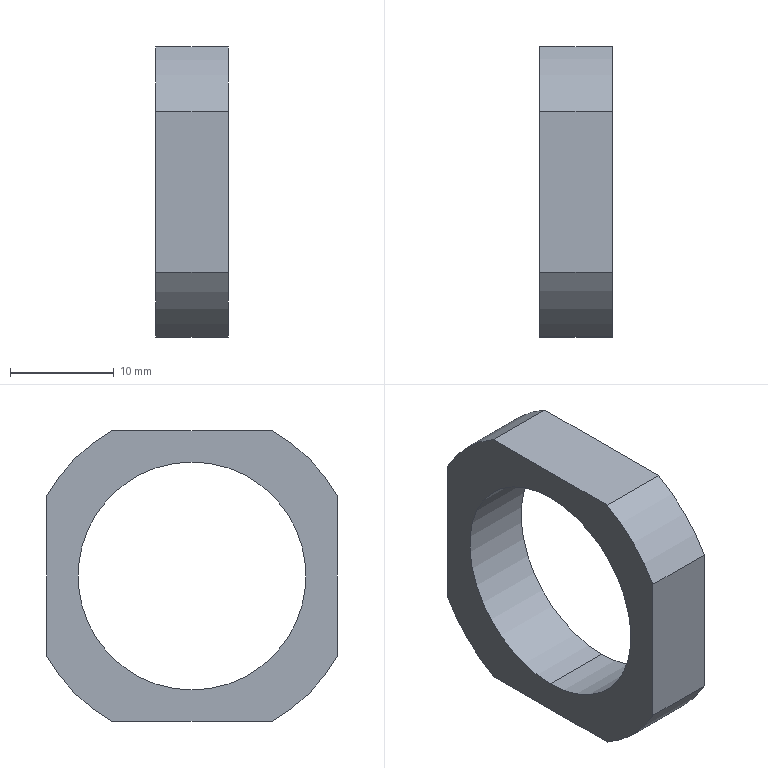Component | SolidWorks | CTM-HVS-42-02-28-1 | 1 solid | 12 faces | box 7 x 28 x 28 mm | volume 2383 mm3 | cylinder 6 | plane 6 | commonest cylinder face diameters 32 x4 22 x2 | material Q235A
build123d program:
from build123d import *

# Parameters (mm, degrees)
SKETCH1_R              = 16
BOSS_EXTRUDE1_DEPTH    = 7
M22X1_5_TAPPED_HOLE1_D = 22
SKETCH2_OUTSIDE_W      = 43.158
SKETCH2_OUTSIDE_H      = 43.158
SKETCH2_OUTSIDE_W_2    = 28
SKETCH2_OUTSIDE_H_2    = 28
CUT_EXTRUDE1_DEPTH     = 7


with BuildPart() as part:
    # Sketch1 → Boss-Extrude1 (new body)
    with BuildSketch(Plane(origin=(0, 0, 0), x_dir=(0, 0, -1), z_dir=(1, 0, 0))):
        Circle(SKETCH1_R)
    extrude(amount=BOSS_EXTRUDE1_DEPTH)

    # M22x1.5 Tapped Hole1 (through all)
    with Locations(Plane(origin=(7, 0, 0), x_dir=(0, 0, -1), z_dir=(1, 0, 0))):
        with Locations((0, 0)):
            Hole(M22X1_5_TAPPED_HOLE1_D / 2)

    # Sketch2 outside → Cut-Extrude1 (cut)
    with BuildSketch(Plane(origin=(7, 0, 0), x_dir=(0, 0, -1), z_dir=(1, 0, 0))):
        Rectangle(SKETCH2_OUTSIDE_W, SKETCH2_OUTSIDE_H)
        Rectangle(SKETCH2_OUTSIDE_W_2, SKETCH2_OUTSIDE_H_2, mode=Mode.SUBTRACT)
    extrude(amount=-CUT_EXTRUDE1_DEPTH, mode=Mode.SUBTRACT)


solid = part.part

# Placed as in the assembly
solid = solid.moved(Location((-307.307, 55.443, 30), (0, 0, 0)))
STEP:
#1=COLOUR_RGB('',0.7922,0.8196,0.9333);
#2=FILL_AREA_STYLE_COLOUR('',#1);
#3=FILL_AREA_STYLE('',(#2));
#4=SURFACE_STYLE_FILL_AREA(#3);
#5=SURFACE_SIDE_STYLE('',(#4));
#6=SURFACE_STYLE_USAGE(.BOTH.,#5);
#7=PRESENTATION_STYLE_ASSIGNMENT((#6));
#8=CARTESIAN_POINT('',(-12.099,2.183,1.614));
#9=VERTEX_POINT('',#8);
#10=CARTESIAN_POINT('',(-12.099,2.183,0.748));
#11=VERTEX_POINT('',#10);
#12=CARTESIAN_POINT('',(-12.099,2.183,1.181));
#13=DIRECTION('',(1.,0.,0.));
#14=DIRECTION('',(0.,0.,-1.));
#15=AXIS2_PLACEMENT_3D('',#12,#13,#14);
#16=CIRCLE('',#15,0.4331);
#17=EDGE_CURVE('',#9,#11,#16,.T.);
#18=ORIENTED_EDGE('',*,*,#17,.F.);
#19=CARTESIAN_POINT('',(-11.823,2.183,1.614));
#20=VERTEX_POINT('',#19);
#21=CARTESIAN_POINT('',(-11.823,2.183,1.614));
#22=DIRECTION('',(1.,0.,0.));
#23=VECTOR('',#22,39.37);
#24=LINE('',#21,#23);
#25=EDGE_CURVE('',#9,#20,#24,.T.);
#26=ORIENTED_EDGE('',*,*,#25,.T.);
#27=CARTESIAN_POINT('',(-11.823,2.183,0.748));
#28=VERTEX_POINT('',#27);
#29=CARTESIAN_POINT('',(-11.823,2.183,1.181));
#30=DIRECTION('',(1.,0.,0.));
#31=DIRECTION('',(0.,0.,-1.));
#32=AXIS2_PLACEMENT_3D('',#29,#30,#31);
#33=CIRCLE('',#32,0.4331);
#34=EDGE_CURVE('',#20,#28,#33,.T.);
#35=ORIENTED_EDGE('',*,*,#34,.T.);
#36=CARTESIAN_POINT('',(-11.823,2.183,0.748));
#37=DIRECTION('',(1.,0.,0.));
#38=VECTOR('',#37,39.37);
#39=LINE('',#36,#38);
#40=EDGE_CURVE('',#11,#28,#39,.T.);
#41=ORIENTED_EDGE('',*,*,#40,.F.);
#42=EDGE_LOOP('',(#18,#26,#35,#41));
#43=FACE_OUTER_BOUND('',#42,.T.);
#44=CARTESIAN_POINT('',(-11.823,2.183,1.181));
#45=DIRECTION('',(1.,0.,0.));
#46=DIRECTION('',(0.,0.,-1.));
#47=AXIS2_PLACEMENT_3D('',#44,#45,#46);
#48=CYLINDRICAL_SURFACE('',#47,0.4331);
#49=ADVANCED_FACE('',(#43),#48,.F.);
#50=CARTESIAN_POINT('',(-12.099,1.878,0.6299));
#51=VERTEX_POINT('',#50);
#52=CARTESIAN_POINT('',(-11.823,1.878,0.6299));
#53=VERTEX_POINT('',#52);
#54=CARTESIAN_POINT('',(-11.823,1.878,0.6299));
#55=DIRECTION('',(1.,0.,0.));
#56=VECTOR('',#55,39.37);
#57=LINE('',#54,#56);
#58=EDGE_CURVE('',#51,#53,#57,.T.);
#59=ORIENTED_EDGE('',*,*,#58,.T.);
#60=CARTESIAN_POINT('',(-11.823,1.632,0.8761));
#61=VERTEX_POINT('',#60);
#62=CARTESIAN_POINT('',(-11.823,2.183,1.181));
#63=DIRECTION('',(1.,0.,0.));
#64=DIRECTION('',(0.,0.,-1.));
#65=AXIS2_PLACEMENT_3D('',#62,#63,#64);
#66=CIRCLE('',#65,0.6299);
#67=EDGE_CURVE('',#61,#53,#66,.T.);
#68=ORIENTED_EDGE('',*,*,#67,.F.);
#69=CARTESIAN_POINT('',(-12.099,1.632,0.8761));
#70=VERTEX_POINT('',#69);
#71=CARTESIAN_POINT('',(-11.823,1.632,0.8761));
#72=DIRECTION('',(-1.,0.,0.));
#73=VECTOR('',#72,39.37);
#74=LINE('',#71,#73);
#75=EDGE_CURVE('',#61,#70,#74,.T.);
#76=ORIENTED_EDGE('',*,*,#75,.T.);
#77=CARTESIAN_POINT('',(-12.099,2.183,1.181));
#78=DIRECTION('',(1.,0.,0.));
#79=DIRECTION('',(0.,0.,-1.));
#80=AXIS2_PLACEMENT_3D('',#77,#78,#79);
#81=CIRCLE('',#80,0.6299);
#82=EDGE_CURVE('',#70,#51,#81,.T.);
#83=ORIENTED_EDGE('',*,*,#82,.T.);
#84=EDGE_LOOP('',(#59,#68,#76,#83));
#85=FACE_OUTER_BOUND('',#84,.T.);
#86=CARTESIAN_POINT('',(-11.823,2.183,1.181));
#87=DIRECTION('',(-1.,0.,0.));
#88=DIRECTION('',(0.,0.,1.));
#89=AXIS2_PLACEMENT_3D('',#86,#87,#88);
#90=CYLINDRICAL_SURFACE('',#89,0.6299);
#91=ADVANCED_FACE('',(#85),#90,.T.);
#92=CARTESIAN_POINT('',(-12.099,1.632,1.486));
#93=VERTEX_POINT('',#92);
#94=CARTESIAN_POINT('',(-11.823,1.632,1.486));
#95=VERTEX_POINT('',#94);
#96=CARTESIAN_POINT('',(-11.823,1.632,1.486));
#97=DIRECTION('',(1.,0.,0.));
#98=VECTOR('',#97,39.37);
#99=LINE('',#96,#98);
#100=EDGE_CURVE('',#93,#95,#99,.T.);
#101=ORIENTED_EDGE('',*,*,#100,.T.);
#102=CARTESIAN_POINT('',(-11.823,1.878,1.732));
#103=VERTEX_POINT('',#102);
#104=CARTESIAN_POINT('',(-11.823,2.183,1.181));
#105=DIRECTION('',(1.,0.,0.));
#106=DIRECTION('',(0.,0.,-1.));
#107=AXIS2_PLACEMENT_3D('',#104,#105,#106);
#108=CIRCLE('',#107,0.6299);
#109=EDGE_CURVE('',#103,#95,#108,.T.);
#110=ORIENTED_EDGE('',*,*,#109,.F.);
#111=CARTESIAN_POINT('',(-12.099,1.878,1.732));
#112=VERTEX_POINT('',#111);
#113=CARTESIAN_POINT('',(-11.823,1.878,1.732));
#114=DIRECTION('',(-1.,0.,0.));
#115=VECTOR('',#114,39.37);
#116=LINE('',#113,#115);
#117=EDGE_CURVE('',#103,#112,#116,.T.);
#118=ORIENTED_EDGE('',*,*,#117,.T.);
#119=CARTESIAN_POINT('',(-12.099,2.183,1.181));
#120=DIRECTION('',(1.,0.,0.));
#121=DIRECTION('',(0.,0.,-1.));
#122=AXIS2_PLACEMENT_3D('',#119,#120,#121);
#123=CIRCLE('',#122,0.6299);
#124=EDGE_CURVE('',#112,#93,#123,.T.);
#125=ORIENTED_EDGE('',*,*,#124,.T.);
#126=EDGE_LOOP('',(#101,#110,#118,#125));
#127=FACE_OUTER_BOUND('',#126,.T.);
#128=CARTESIAN_POINT('',(-11.823,2.183,1.181));
#129=DIRECTION('',(-1.,0.,0.));
#130=DIRECTION('',(0.,0.,1.));
#131=AXIS2_PLACEMENT_3D('',#128,#129,#130);
#132=CYLINDRICAL_SURFACE('',#131,0.6299);
#133=ADVANCED_FACE('',(#127),#132,.T.);
#134=CARTESIAN_POINT('',(-12.099,2.488,1.732));
#135=VERTEX_POINT('',#134);
#136=CARTESIAN_POINT('',(-11.823,2.488,1.732));
#137=VERTEX_POINT('',#136);
#138=CARTESIAN_POINT('',(-11.823,2.488,1.732));
#139=DIRECTION('',(1.,0.,0.));
#140=VECTOR('',#139,39.37);
#141=LINE('',#138,#140);
#142=EDGE_CURVE('',#135,#137,#141,.T.);
#143=ORIENTED_EDGE('',*,*,#142,.T.);
#144=CARTESIAN_POINT('',(-11.823,2.734,1.486));
#145=VERTEX_POINT('',#144);
#146=CARTESIAN_POINT('',(-11.823,2.183,1.181));
#147=DIRECTION('',(1.,0.,0.));
#148=DIRECTION('',(0.,0.,-1.));
#149=AXIS2_PLACEMENT_3D('',#146,#147,#148);
#150=CIRCLE('',#149,0.6299);
#151=EDGE_CURVE('',#145,#137,#150,.T.);
#152=ORIENTED_EDGE('',*,*,#151,.F.);
#153=CARTESIAN_POINT('',(-12.099,2.734,1.486));
#154=VERTEX_POINT('',#153);
#155=CARTESIAN_POINT('',(-11.823,2.734,1.486));
#156=DIRECTION('',(-1.,0.,0.));
#157=VECTOR('',#156,39.37);
#158=LINE('',#155,#157);
#159=EDGE_CURVE('',#145,#154,#158,.T.);
#160=ORIENTED_EDGE('',*,*,#159,.T.);
#161=CARTESIAN_POINT('',(-12.099,2.183,1.181));
#162=DIRECTION('',(1.,0.,0.));
#163=DIRECTION('',(0.,0.,-1.));
#164=AXIS2_PLACEMENT_3D('',#161,#162,#163);
#165=CIRCLE('',#164,0.6299);
#166=EDGE_CURVE('',#154,#135,#165,.T.);
#167=ORIENTED_EDGE('',*,*,#166,.T.);
#168=EDGE_LOOP('',(#143,#152,#160,#167));
#169=FACE_OUTER_BOUND('',#168,.T.);
#170=CARTESIAN_POINT('',(-11.823,2.183,1.181));
#171=DIRECTION('',(-1.,0.,0.));
#172=DIRECTION('',(0.,0.,1.));
#173=AXIS2_PLACEMENT_3D('',#170,#171,#172);
#174=CYLINDRICAL_SURFACE('',#173,0.6299);
#175=ADVANCED_FACE('',(#169),#174,.T.);
#176=CARTESIAN_POINT('',(-11.823,2.488,0.6299));
#177=VERTEX_POINT('',#176);
#178=CARTESIAN_POINT('',(-12.099,2.488,0.6299));
#179=VERTEX_POINT('',#178);
#180=CARTESIAN_POINT('',(-11.823,2.488,0.6299));
#181=DIRECTION('',(-1.,0.,0.));
#182=VECTOR('',#181,39.37);
#183=LINE('',#180,#182);
#184=EDGE_CURVE('',#177,#179,#183,.T.);
#185=ORIENTED_EDGE('',*,*,#184,.T.);
#186=CARTESIAN_POINT('',(-12.099,2.734,0.8761));
#187=VERTEX_POINT('',#186);
#188=CARTESIAN_POINT('',(-12.099,2.183,1.181));
#189=DIRECTION('',(1.,0.,0.));
#190=DIRECTION('',(0.,0.,-1.));
#191=AXIS2_PLACEMENT_3D('',#188,#189,#190);
#192=CIRCLE('',#191,0.6299);
#193=EDGE_CURVE('',#179,#187,#192,.T.);
#194=ORIENTED_EDGE('',*,*,#193,.T.);
#195=CARTESIAN_POINT('',(-11.823,2.734,0.8761));
#196=VERTEX_POINT('',#195);
#197=CARTESIAN_POINT('',(-11.823,2.734,0.8761));
#198=DIRECTION('',(1.,0.,0.));
#199=VECTOR('',#198,39.37);
#200=LINE('',#197,#199);
#201=EDGE_CURVE('',#187,#196,#200,.T.);
#202=ORIENTED_EDGE('',*,*,#201,.T.);
#203=CARTESIAN_POINT('',(-11.823,2.183,1.181));
#204=DIRECTION('',(1.,0.,0.));
#205=DIRECTION('',(0.,0.,-1.));
#206=AXIS2_PLACEMENT_3D('',#203,#204,#205);
#207=CIRCLE('',#206,0.6299);
#208=EDGE_CURVE('',#177,#196,#207,.T.);
#209=ORIENTED_EDGE('',*,*,#208,.F.);
#210=EDGE_LOOP('',(#185,#194,#202,#209));
#211=FACE_OUTER_BOUND('',#210,.T.);
#212=CARTESIAN_POINT('',(-11.823,2.183,1.181));
#213=DIRECTION('',(-1.,0.,0.));
#214=DIRECTION('',(0.,0.,1.));
#215=AXIS2_PLACEMENT_3D('',#212,#213,#214);
#216=CYLINDRICAL_SURFACE('',#215,0.6299);
#217=ADVANCED_FACE('',(#211),#216,.T.);
#218=CARTESIAN_POINT('',(-11.823,2.183,1.181));
#219=DIRECTION('',(1.,0.,0.));
#220=DIRECTION('',(0.,0.,-1.));
#221=AXIS2_PLACEMENT_3D('',#218,#219,#220);
#222=CIRCLE('',#221,0.4331);
#223=EDGE_CURVE('',#28,#20,#222,.T.);
#224=ORIENTED_EDGE('',*,*,#223,.F.);
#225=ORIENTED_EDGE('',*,*,#34,.F.);
#226=EDGE_LOOP('',(#224,#225));
#227=FACE_BOUND('',#226,.T.);
#228=ORIENTED_EDGE('',*,*,#67,.T.);
#229=CARTESIAN_POINT('',(-11.823,1.632,0.6299));
#230=DIRECTION('',(0.,1.,0.));
#231=VECTOR('',#230,39.37);
#232=LINE('',#229,#231);
#233=EDGE_CURVE('',#53,#177,#232,.T.);
#234=ORIENTED_EDGE('',*,*,#233,.T.);
#235=ORIENTED_EDGE('',*,*,#208,.T.);
#236=CARTESIAN_POINT('',(-11.823,2.734,1.732));
#237=DIRECTION('',(0.,0.,1.));
#238=VECTOR('',#237,39.37);
#239=LINE('',#236,#238);
#240=EDGE_CURVE('',#196,#145,#239,.T.);
#241=ORIENTED_EDGE('',*,*,#240,.T.);
#242=ORIENTED_EDGE('',*,*,#151,.T.);
#243=CARTESIAN_POINT('',(-11.823,1.632,1.732));
#244=DIRECTION('',(0.,-1.,0.));
#245=VECTOR('',#244,39.37);
#246=LINE('',#243,#245);
#247=EDGE_CURVE('',#137,#103,#246,.T.);
#248=ORIENTED_EDGE('',*,*,#247,.T.);
#249=ORIENTED_EDGE('',*,*,#109,.T.);
#250=CARTESIAN_POINT('',(-11.823,1.632,1.732));
#251=DIRECTION('',(0.,0.,-1.));
#252=VECTOR('',#251,39.37);
#253=LINE('',#250,#252);
#254=EDGE_CURVE('',#95,#61,#253,.T.);
#255=ORIENTED_EDGE('',*,*,#254,.T.);
#256=EDGE_LOOP('',(#228,#234,#235,#241,#242,#248,#249,#255));
#257=FACE_OUTER_BOUND('',#256,.T.);
#258=CARTESIAN_POINT('',(-11.823,2.183,1.181));
#259=DIRECTION('',(1.,0.,0.));
#260=DIRECTION('',(0.,0.,-1.));
#261=AXIS2_PLACEMENT_3D('',#258,#259,#260);
#262=PLANE('',#261);
#263=ADVANCED_FACE('',(#227,#257),#262,.T.);
#264=CARTESIAN_POINT('',(-12.099,1.632,0.6299));
#265=DIRECTION('',(0.,-1.,0.));
#266=VECTOR('',#265,39.37);
#267=LINE('',#264,#266);
#268=EDGE_CURVE('',#179,#51,#267,.T.);
#269=ORIENTED_EDGE('',*,*,#268,.T.);
#270=ORIENTED_EDGE('',*,*,#82,.F.);
#271=CARTESIAN_POINT('',(-12.099,1.632,1.732));
#272=DIRECTION('',(0.,0.,1.));
#273=VECTOR('',#272,39.37);
#274=LINE('',#271,#273);
#275=EDGE_CURVE('',#70,#93,#274,.T.);
#276=ORIENTED_EDGE('',*,*,#275,.T.);
#277=ORIENTED_EDGE('',*,*,#124,.F.);
#278=CARTESIAN_POINT('',(-12.099,1.632,1.732));
#279=DIRECTION('',(0.,1.,0.));
#280=VECTOR('',#279,39.37);
#281=LINE('',#278,#280);
#282=EDGE_CURVE('',#112,#135,#281,.T.);
#283=ORIENTED_EDGE('',*,*,#282,.T.);
#284=ORIENTED_EDGE('',*,*,#166,.F.);
#285=CARTESIAN_POINT('',(-12.099,2.734,1.732));
#286=DIRECTION('',(0.,0.,-1.));
#287=VECTOR('',#286,39.37);
#288=LINE('',#285,#287);
#289=EDGE_CURVE('',#154,#187,#288,.T.);
#290=ORIENTED_EDGE('',*,*,#289,.T.);
#291=ORIENTED_EDGE('',*,*,#193,.F.);
#292=EDGE_LOOP('',(#269,#270,#276,#277,#283,#284,#290,#291));
#293=FACE_OUTER_BOUND('',#292,.T.);
#294=CARTESIAN_POINT('',(-12.099,2.183,1.181));
#295=DIRECTION('',(1.,0.,0.));
#296=DIRECTION('',(0.,0.,-1.));
#297=AXIS2_PLACEMENT_3D('',#294,#295,#296);
#298=CIRCLE('',#297,0.4331);
#299=EDGE_CURVE('',#11,#9,#298,.T.);
#300=ORIENTED_EDGE('',*,*,#299,.T.);
#301=ORIENTED_EDGE('',*,*,#17,.T.);
#302=EDGE_LOOP('',(#300,#301));
#303=FACE_BOUND('',#302,.T.);
#304=CARTESIAN_POINT('',(-12.099,2.183,1.181));
#305=DIRECTION('',(1.,0.,0.));
#306=DIRECTION('',(0.,0.,-1.));
#307=AXIS2_PLACEMENT_3D('',#304,#305,#306);
#308=PLANE('',#307);
#309=ADVANCED_FACE('',(#293,#303),#308,.F.);
#310=ORIENTED_EDGE('',*,*,#25,.F.);
#311=ORIENTED_EDGE('',*,*,#299,.F.);
#312=ORIENTED_EDGE('',*,*,#40,.T.);
#313=ORIENTED_EDGE('',*,*,#223,.T.);
#314=EDGE_LOOP('',(#310,#311,#312,#313));
#315=FACE_OUTER_BOUND('',#314,.T.);
#316=CARTESIAN_POINT('',(-11.823,2.183,1.181));
#317=DIRECTION('',(1.,0.,0.));
#318=DIRECTION('',(0.,0.,-1.));
#319=AXIS2_PLACEMENT_3D('',#316,#317,#318);
#320=CYLINDRICAL_SURFACE('',#319,0.4331);
#321=ADVANCED_FACE('',(#315),#320,.F.);
#322=ORIENTED_EDGE('',*,*,#201,.F.);
#323=ORIENTED_EDGE('',*,*,#289,.F.);
#324=ORIENTED_EDGE('',*,*,#159,.F.);
#325=ORIENTED_EDGE('',*,*,#240,.F.);
#326=EDGE_LOOP('',(#322,#323,#324,#325));
#327=FACE_OUTER_BOUND('',#326,.T.);
#328=CARTESIAN_POINT('',(-12.099,2.734,1.732));
#329=DIRECTION('',(0.,1.,0.));
#330=DIRECTION('',(0.,0.,1.));
#331=AXIS2_PLACEMENT_3D('',#328,#329,#330);
#332=PLANE('',#331);
#333=ADVANCED_FACE('',(#327),#332,.T.);
#334=ORIENTED_EDGE('',*,*,#142,.F.);
#335=ORIENTED_EDGE('',*,*,#282,.F.);
#336=ORIENTED_EDGE('',*,*,#117,.F.);
#337=ORIENTED_EDGE('',*,*,#247,.F.);
#338=EDGE_LOOP('',(#334,#335,#336,#337));
#339=FACE_OUTER_BOUND('',#338,.T.);
#340=CARTESIAN_POINT('',(-12.099,1.632,1.732));
#341=DIRECTION('',(0.,0.,1.));
#342=DIRECTION('',(1.,0.,0.));
#343=AXIS2_PLACEMENT_3D('',#340,#341,#342);
#344=PLANE('',#343);
#345=ADVANCED_FACE('',(#339),#344,.T.);
#346=ORIENTED_EDGE('',*,*,#100,.F.);
#347=ORIENTED_EDGE('',*,*,#275,.F.);
#348=ORIENTED_EDGE('',*,*,#75,.F.);
#349=ORIENTED_EDGE('',*,*,#254,.F.);
#350=EDGE_LOOP('',(#346,#347,#348,#349));
#351=FACE_OUTER_BOUND('',#350,.T.);
#352=CARTESIAN_POINT('',(-12.099,1.632,1.732));
#353=DIRECTION('',(0.,-1.,0.));
#354=DIRECTION('',(0.,0.,-1.));
#355=AXIS2_PLACEMENT_3D('',#352,#353,#354);
#356=PLANE('',#355);
#357=ADVANCED_FACE('',(#351),#356,.T.);
#358=ORIENTED_EDGE('',*,*,#58,.F.);
#359=ORIENTED_EDGE('',*,*,#268,.F.);
#360=ORIENTED_EDGE('',*,*,#184,.F.);
#361=ORIENTED_EDGE('',*,*,#233,.F.);
#362=EDGE_LOOP('',(#358,#359,#360,#361));
#363=FACE_OUTER_BOUND('',#362,.T.);
#364=CARTESIAN_POINT('',(-12.099,1.632,0.6299));
#365=DIRECTION('',(0.,0.,-1.));
#366=DIRECTION('',(-1.,0.,0.));
#367=AXIS2_PLACEMENT_3D('',#364,#365,#366);
#368=PLANE('',#367);
#369=ADVANCED_FACE('',(#363),#368,.T.);
#370=CLOSED_SHELL('',(#49,#91,#133,#175,#217,#263,#309,#321,#333,#345,#357,#369));
#371=MANIFOLD_SOLID_BREP('',#370);
#372=STYLED_ITEM('',(#7),#371);
#373=(LENGTH_UNIT()NAMED_UNIT(*)SI_UNIT($,.METRE.));
#374=LENGTH_MEASURE_WITH_UNIT(LENGTH_MEASURE(0.0254),#373);
#375=DIMENSIONAL_EXPONENTS(1.,0.,0.,0.,0.,0.,0.);
#376=(CONVERSION_BASED_UNIT('',#374)LENGTH_UNIT()NAMED_UNIT(#375));
#377=UNCERTAINTY_MEASURE_WITH_UNIT(LENGTH_MEASURE(0.00001),#376,'','');
#378=(NAMED_UNIT(*)PLANE_ANGLE_UNIT()SI_UNIT($,.RADIAN.));
#379=(NAMED_UNIT(*)SI_UNIT($,.STERADIAN.)SOLID_ANGLE_UNIT());
#380=(GEOMETRIC_REPRESENTATION_CONTEXT(3)GLOBAL_UNCERTAINTY_ASSIGNED_CONTEXT((#377))GLOBAL_UNIT_ASSIGNED_CONTEXT((#376,#378,#379))REPRESENTATION_CONTEXT('',''));
#381=MECHANICAL_DESIGN_GEOMETRIC_PRESENTATION_REPRESENTATION('',(#372),#380);
#382=CARTESIAN_POINT('',(0.,0.,0.));
#383=DIRECTION('',(0.,0.,1.));
#384=DIRECTION('',(1.,0.,0.));
#385=AXIS2_PLACEMENT_3D('',#382,#383,#384);
#386=(LENGTH_UNIT()NAMED_UNIT(*)SI_UNIT($,.METRE.));
#387=LENGTH_MEASURE_WITH_UNIT(LENGTH_MEASURE(0.0254),#386);
#388=DIMENSIONAL_EXPONENTS(1.,0.,0.,0.,0.,0.,0.);
#389=(CONVERSION_BASED_UNIT('',#387)LENGTH_UNIT()NAMED_UNIT(#388));
#390=UNCERTAINTY_MEASURE_WITH_UNIT(LENGTH_MEASURE(0.00001),#389,'','');
#391=(NAMED_UNIT(*)PLANE_ANGLE_UNIT()SI_UNIT($,.RADIAN.));
#392=(NAMED_UNIT(*)SI_UNIT($,.STERADIAN.)SOLID_ANGLE_UNIT());
#393=(GEOMETRIC_REPRESENTATION_CONTEXT(3)GLOBAL_UNCERTAINTY_ASSIGNED_CONTEXT((#390))GLOBAL_UNIT_ASSIGNED_CONTEXT((#389,#391,#392))REPRESENTATION_CONTEXT('',''));
#394=ADVANCED_BREP_SHAPE_REPRESENTATION('',(#371,#385),#393);
#395=PRESENTATION_LAYER_ASSIGNMENT('','',(#372));